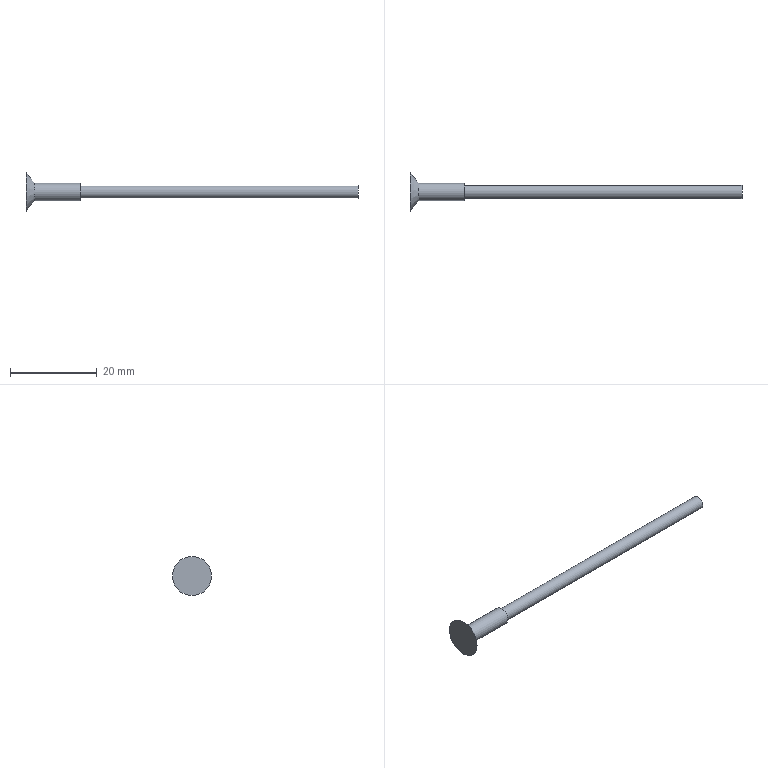Component | NX | LINK_4 | 1 solid | 6 faces | volume 654 mm3 | plane 3 | cylinder 2 | cone 1 | commonest cylinder face diameters 3 x1 4 x1